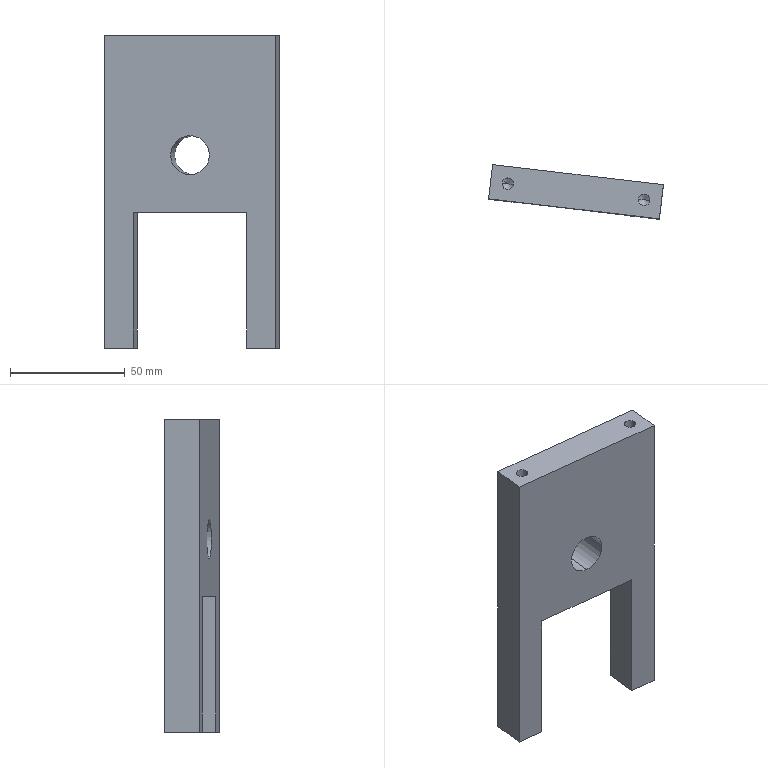Component | SolidWorks | 8TC-A17001-90-01PressureRollerSidePlate1-1 | 1 solid | 28 faces | box 76.24 x 23.65 x 136.2 mm | volume 103614 mm3 | cylinder 10 | plane 10 | cone 8 | commonest cylinder face diameters 5 x8 17 x2 | material #45
build123d program:
from build123d import *

# Parameters (mm, degrees)
SKETCH1_W                  = 75
SKETCH1_H                  = 77
BOSS_EXTRUDE1_DEPTH        = 7.5
SKETCH23_W                 = 12.5
SKETCH23_H                 = 15
BOSS_EXTRUDE4_DEPTH        = 59.2
M6_TAPPED_HOLE2_D          = 5
M6_TAPPED_HOLE2_DEPTH      = 25
M6_TAPPED_HOLE2_TIP        = 1.502
M6_TAPPED_HOLE1_D          = 5
M6_TAPPED_HOLE1_DEPTH      = 20
M6_TAPPED_HOLE1_TIP        = 1.502
F_15_0_15_DIAMETER_HOLE1_D = 17


with BuildPart() as part:
    # Sketch1 → Boss-Extrude1 (new, symmetric)
    with BuildSketch(Plane(origin=(0, 0, 0), x_dir=(1, 0, 0), z_dir=(0, 1, 0))):
        Rectangle(SKETCH1_W, SKETCH1_H)
    extrude(amount=BOSS_EXTRUDE1_DEPTH, both=True)

    # Sketch23 → Boss-Extrude4 (add)
    with BuildSketch(Plane.XY.offset(38.5)):
        with Locations((-31.25, 0)):
            Rectangle(SKETCH23_W, SKETCH23_H)
        with Locations((31.25, 0)):
            Rectangle(SKETCH23_W, SKETCH23_H)
    extrude(amount=BOSS_EXTRUDE4_DEPTH)

    # M6 Tapped Hole2
    with Locations(Plane.XY.offset(97.7)):
        with Locations((-30, 0), (30, 0)):
            Hole(M6_TAPPED_HOLE2_D / 2, depth=M6_TAPPED_HOLE2_DEPTH)
            with Locations((0, 0, -(M6_TAPPED_HOLE2_DEPTH + M6_TAPPED_HOLE2_TIP / 2))):  # 118° drill point
                Cone(0, M6_TAPPED_HOLE2_D / 2, M6_TAPPED_HOLE2_TIP, mode=Mode.SUBTRACT)

    # M6 Tapped Hole1
    with Locations(Plane(origin=(0, 0, -38.5), x_dir=(-1, 0, 0), z_dir=(0, 0, -1))):
        with Locations((-30, 0), (30, 0)):
            Hole(M6_TAPPED_HOLE1_D / 2, depth=M6_TAPPED_HOLE1_DEPTH)
            with Locations((0, 0, -(M6_TAPPED_HOLE1_DEPTH + M6_TAPPED_HOLE1_TIP / 2))):  # 118° drill point
                Cone(0, M6_TAPPED_HOLE1_D / 2, M6_TAPPED_HOLE1_TIP, mode=Mode.SUBTRACT)

    # 15.0 _15_ Diameter Hole1 (through all)
    with Locations(Plane(origin=(0, 7.5, 0), x_dir=(1, 0, 0), z_dir=(0, 1, 0))):
        with Locations((0, -13.5)):
            Hole(F_15_0_15_DIAMETER_HOLE1_D / 2)


solid = part.part

# Placed as in the assembly
solid = solid.moved(Location((-0.2049, -94, -38.5), (-180, 0, -173.3)))
STEP:
#1=COLOUR_RGB('',0.7922,0.8196,0.9333);
#2=FILL_AREA_STYLE_COLOUR('',#1);
#3=FILL_AREA_STYLE('',(#2));
#4=SURFACE_STYLE_FILL_AREA(#3);
#5=SURFACE_SIDE_STYLE('',(#4));
#6=SURFACE_STYLE_USAGE(.BOTH.,#5);
#7=PRESENTATION_STYLE_ASSIGNMENT((#6));
#8=CARTESIAN_POINT('',(-0.04251,-3.994,-1.713));
#9=VERTEX_POINT('',#8);
#10=CARTESIAN_POINT('',(-0.04251,-3.994,-2.382));
#11=VERTEX_POINT('',#10);
#12=CARTESIAN_POINT('',(-0.04251,-3.994,-2.047));
#13=DIRECTION('',(0.1167,0.9932,-0.));
#14=DIRECTION('',(0.,0.,-1.));
#15=AXIS2_PLACEMENT_3D('',#12,#13,#14);
#16=CIRCLE('',#15,0.3346);
#17=EDGE_CURVE('',#9,#11,#16,.T.);
#18=ORIENTED_EDGE('',*,*,#17,.F.);
#19=CARTESIAN_POINT('',(0.02638,-3.408,-1.713));
#20=VERTEX_POINT('',#19);
#21=CARTESIAN_POINT('',(0.02638,-3.408,-1.713));
#22=DIRECTION('',(0.1167,0.9932,-0.));
#23=VECTOR('',#22,39.37);
#24=LINE('',#21,#23);
#25=EDGE_CURVE('',#9,#20,#24,.T.);
#26=ORIENTED_EDGE('',*,*,#25,.T.);
#27=CARTESIAN_POINT('',(0.02638,-3.408,-2.382));
#28=VERTEX_POINT('',#27);
#29=CARTESIAN_POINT('',(0.02638,-3.408,-2.047));
#30=DIRECTION('',(0.1167,0.9932,-0.));
#31=DIRECTION('',(0.,0.,-1.));
#32=AXIS2_PLACEMENT_3D('',#29,#30,#31);
#33=CIRCLE('',#32,0.3346);
#34=EDGE_CURVE('',#20,#28,#33,.T.);
#35=ORIENTED_EDGE('',*,*,#34,.T.);
#36=CARTESIAN_POINT('',(0.02638,-3.408,-2.382));
#37=DIRECTION('',(0.1167,0.9932,-0.));
#38=VECTOR('',#37,39.37);
#39=LINE('',#36,#38);
#40=EDGE_CURVE('',#11,#28,#39,.T.);
#41=ORIENTED_EDGE('',*,*,#40,.F.);
#42=EDGE_LOOP('',(#18,#26,#35,#41));
#43=FACE_OUTER_BOUND('',#42,.T.);
#44=CARTESIAN_POINT('',(0.02638,-3.408,-2.047));
#45=DIRECTION('',(0.1167,0.9932,-0.));
#46=DIRECTION('',(0.,0.,-1.));
#47=AXIS2_PLACEMENT_3D('',#44,#45,#46);
#48=CYLINDRICAL_SURFACE('',#47,0.3346);
#49=ADVANCED_FACE('',(#43),#48,.F.);
#50=CARTESIAN_POINT('',(-1.279,-3.552,-0.7874));
#51=VERTEX_POINT('',#50);
#52=CARTESIAN_POINT('',(-1.083,-3.574,-0.7874));
#53=VERTEX_POINT('',#52);
#54=CARTESIAN_POINT('',(-1.181,-3.563,-0.7874));
#55=DIRECTION('',(-0.,0.,1.));
#56=DIRECTION('',(0.9932,-0.1167,0.));
#57=AXIS2_PLACEMENT_3D('',#54,#55,#56);
#58=CIRCLE('',#57,0.09843);
#59=EDGE_CURVE('',#51,#53,#58,.T.);
#60=ORIENTED_EDGE('',*,*,#59,.F.);
#61=CARTESIAN_POINT('',(-1.279,-3.552,-0.));
#62=VERTEX_POINT('',#61);
#63=CARTESIAN_POINT('',(-1.279,-3.552,-0.));
#64=DIRECTION('',(-0.,0.,1.));
#65=VECTOR('',#64,39.37);
#66=LINE('',#63,#65);
#67=EDGE_CURVE('',#51,#62,#66,.T.);
#68=ORIENTED_EDGE('',*,*,#67,.T.);
#69=CARTESIAN_POINT('',(-1.083,-3.574,0.));
#70=VERTEX_POINT('',#69);
#71=CARTESIAN_POINT('',(-1.181,-3.563,0.));
#72=DIRECTION('',(-0.,0.,1.));
#73=DIRECTION('',(0.9932,-0.1167,0.));
#74=AXIS2_PLACEMENT_3D('',#71,#72,#73);
#75=CIRCLE('',#74,0.09843);
#76=EDGE_CURVE('',#62,#70,#75,.T.);
#77=ORIENTED_EDGE('',*,*,#76,.T.);
#78=CARTESIAN_POINT('',(-1.083,-3.574,0.));
#79=DIRECTION('',(-0.,0.,1.));
#80=VECTOR('',#79,39.37);
#81=LINE('',#78,#80);
#82=EDGE_CURVE('',#53,#70,#81,.T.);
#83=ORIENTED_EDGE('',*,*,#82,.F.);
#84=EDGE_LOOP('',(#60,#68,#77,#83));
#85=FACE_OUTER_BOUND('',#84,.T.);
#86=CARTESIAN_POINT('',(-1.181,-3.563,0.));
#87=DIRECTION('',(-0.,0.,1.));
#88=DIRECTION('',(0.9932,-0.1167,0.));
#89=AXIS2_PLACEMENT_3D('',#86,#87,#88);
#90=CYLINDRICAL_SURFACE('',#89,0.09843);
#91=ADVANCED_FACE('',(#85),#90,.F.);
#92=CARTESIAN_POINT('',(-1.181,-3.563,-0.8465));
#93=VERTEX_POINT('',#92);
#94=CARTESIAN_POINT('',(-1.083,-3.574,-0.7874));
#95=DIRECTION('',(0.8513,-0.1,0.515));
#96=VECTOR('',#95,39.37);
#97=LINE('',#94,#96);
#98=EDGE_CURVE('',#93,#53,#97,.T.);
#99=ORIENTED_EDGE('',*,*,#98,.F.);
#100=CARTESIAN_POINT('',(-1.279,-3.552,-0.7874));
#101=DIRECTION('',(-0.8513,0.1,0.515));
#102=VECTOR('',#101,39.37);
#103=LINE('',#100,#102);
#104=EDGE_CURVE('',#93,#51,#103,.T.);
#105=ORIENTED_EDGE('',*,*,#104,.T.);
#106=ORIENTED_EDGE('',*,*,#59,.T.);
#107=EDGE_LOOP('',(#99,#105,#106));
#108=FACE_OUTER_BOUND('',#107,.T.);
#109=CARTESIAN_POINT('',(-1.181,-3.563,-0.7874));
#110=DIRECTION('',(-0.,0.,1.));
#111=DIRECTION('',(0.9932,-0.1167,0.));
#112=AXIS2_PLACEMENT_3D('',#109,#110,#111);
#113=CONICAL_SURFACE('',#112,0.09843,1.03);
#114=ADVANCED_FACE('',(#108),#113,.F.);
#115=CARTESIAN_POINT('',(1.067,-3.827,-0.7874));
#116=VERTEX_POINT('',#115);
#117=CARTESIAN_POINT('',(1.263,-3.85,-0.7874));
#118=VERTEX_POINT('',#117);
#119=CARTESIAN_POINT('',(1.165,-3.839,-0.7874));
#120=DIRECTION('',(-0.,0.,1.));
#121=DIRECTION('',(0.9932,-0.1167,0.));
#122=AXIS2_PLACEMENT_3D('',#119,#120,#121);
#123=CIRCLE('',#122,0.09843);
#124=EDGE_CURVE('',#116,#118,#123,.T.);
#125=ORIENTED_EDGE('',*,*,#124,.F.);
#126=CARTESIAN_POINT('',(1.067,-3.827,-0.));
#127=VERTEX_POINT('',#126);
#128=CARTESIAN_POINT('',(1.067,-3.827,-0.));
#129=DIRECTION('',(-0.,0.,1.));
#130=VECTOR('',#129,39.37);
#131=LINE('',#128,#130);
#132=EDGE_CURVE('',#116,#127,#131,.T.);
#133=ORIENTED_EDGE('',*,*,#132,.T.);
#134=CARTESIAN_POINT('',(1.263,-3.85,0.));
#135=VERTEX_POINT('',#134);
#136=CARTESIAN_POINT('',(1.165,-3.839,0.));
#137=DIRECTION('',(-0.,0.,1.));
#138=DIRECTION('',(0.9932,-0.1167,0.));
#139=AXIS2_PLACEMENT_3D('',#136,#137,#138);
#140=CIRCLE('',#139,0.09843);
#141=EDGE_CURVE('',#127,#135,#140,.T.);
#142=ORIENTED_EDGE('',*,*,#141,.T.);
#143=CARTESIAN_POINT('',(1.263,-3.85,0.));
#144=DIRECTION('',(-0.,0.,1.));
#145=VECTOR('',#144,39.37);
#146=LINE('',#143,#145);
#147=EDGE_CURVE('',#118,#135,#146,.T.);
#148=ORIENTED_EDGE('',*,*,#147,.F.);
#149=EDGE_LOOP('',(#125,#133,#142,#148));
#150=FACE_OUTER_BOUND('',#149,.T.);
#151=CARTESIAN_POINT('',(1.165,-3.839,0.));
#152=DIRECTION('',(-0.,0.,1.));
#153=DIRECTION('',(0.9932,-0.1167,0.));
#154=AXIS2_PLACEMENT_3D('',#151,#152,#153);
#155=CYLINDRICAL_SURFACE('',#154,0.09843);
#156=ADVANCED_FACE('',(#150),#155,.F.);
#157=CARTESIAN_POINT('',(1.165,-3.839,-0.8465));
#158=VERTEX_POINT('',#157);
#159=CARTESIAN_POINT('',(1.263,-3.85,-0.7874));
#160=DIRECTION('',(0.8513,-0.1,0.515));
#161=VECTOR('',#160,39.37);
#162=LINE('',#159,#161);
#163=EDGE_CURVE('',#158,#118,#162,.T.);
#164=ORIENTED_EDGE('',*,*,#163,.F.);
#165=CARTESIAN_POINT('',(1.067,-3.827,-0.7874));
#166=DIRECTION('',(-0.8513,0.1,0.515));
#167=VECTOR('',#166,39.37);
#168=LINE('',#165,#167);
#169=EDGE_CURVE('',#158,#116,#168,.T.);
#170=ORIENTED_EDGE('',*,*,#169,.T.);
#171=ORIENTED_EDGE('',*,*,#124,.T.);
#172=EDGE_LOOP('',(#164,#170,#171));
#173=FACE_OUTER_BOUND('',#172,.T.);
#174=CARTESIAN_POINT('',(1.165,-3.839,-0.7874));
#175=DIRECTION('',(-0.,0.,1.));
#176=DIRECTION('',(0.9932,-0.1167,0.));
#177=AXIS2_PLACEMENT_3D('',#174,#175,#176);
#178=CONICAL_SURFACE('',#177,0.09843,1.03);
#179=ADVANCED_FACE('',(#173),#178,.F.);
#180=CARTESIAN_POINT('',(1.263,-3.85,-4.378));
#181=VERTEX_POINT('',#180);
#182=CARTESIAN_POINT('',(1.067,-3.827,-4.378));
#183=VERTEX_POINT('',#182);
#184=CARTESIAN_POINT('',(1.165,-3.839,-4.378));
#185=DIRECTION('',(0.,-0.,-1.));
#186=DIRECTION('',(-0.9932,0.1167,0.));
#187=AXIS2_PLACEMENT_3D('',#184,#185,#186);
#188=CIRCLE('',#187,0.09843);
#189=EDGE_CURVE('',#181,#183,#188,.T.);
#190=ORIENTED_EDGE('',*,*,#189,.F.);
#191=CARTESIAN_POINT('',(1.263,-3.85,-5.362));
#192=VERTEX_POINT('',#191);
#193=CARTESIAN_POINT('',(1.263,-3.85,-5.362));
#194=DIRECTION('',(0.,-0.,-1.));
#195=VECTOR('',#194,39.37);
#196=LINE('',#193,#195);
#197=EDGE_CURVE('',#181,#192,#196,.T.);
#198=ORIENTED_EDGE('',*,*,#197,.T.);
#199=CARTESIAN_POINT('',(1.067,-3.827,-5.362));
#200=VERTEX_POINT('',#199);
#201=CARTESIAN_POINT('',(1.165,-3.839,-5.362));
#202=DIRECTION('',(0.,-0.,-1.));
#203=DIRECTION('',(-0.9932,0.1167,0.));
#204=AXIS2_PLACEMENT_3D('',#201,#202,#203);
#205=CIRCLE('',#204,0.09843);
#206=EDGE_CURVE('',#192,#200,#205,.T.);
#207=ORIENTED_EDGE('',*,*,#206,.T.);
#208=CARTESIAN_POINT('',(1.067,-3.827,-5.362));
#209=DIRECTION('',(0.,-0.,-1.));
#210=VECTOR('',#209,39.37);
#211=LINE('',#208,#210);
#212=EDGE_CURVE('',#183,#200,#211,.T.);
#213=ORIENTED_EDGE('',*,*,#212,.F.);
#214=EDGE_LOOP('',(#190,#198,#207,#213));
#215=FACE_OUTER_BOUND('',#214,.T.);
#216=CARTESIAN_POINT('',(1.165,-3.839,-5.362));
#217=DIRECTION('',(0.,-0.,-1.));
#218=DIRECTION('',(-0.9932,0.1167,0.));
#219=AXIS2_PLACEMENT_3D('',#216,#217,#218);
#220=CYLINDRICAL_SURFACE('',#219,0.09843);
#221=ADVANCED_FACE('',(#215),#220,.F.);
#222=CARTESIAN_POINT('',(1.165,-3.839,-4.319));
#223=VERTEX_POINT('',#222);
#224=CARTESIAN_POINT('',(1.067,-3.827,-4.378));
#225=DIRECTION('',(-0.8513,0.1,-0.515));
#226=VECTOR('',#225,39.37);
#227=LINE('',#224,#226);
#228=EDGE_CURVE('',#223,#183,#227,.T.);
#229=ORIENTED_EDGE('',*,*,#228,.F.);
#230=CARTESIAN_POINT('',(1.263,-3.85,-4.378));
#231=DIRECTION('',(0.8513,-0.1,-0.515));
#232=VECTOR('',#231,39.37);
#233=LINE('',#230,#232);
#234=EDGE_CURVE('',#223,#181,#233,.T.);
#235=ORIENTED_EDGE('',*,*,#234,.T.);
#236=ORIENTED_EDGE('',*,*,#189,.T.);
#237=EDGE_LOOP('',(#229,#235,#236));
#238=FACE_OUTER_BOUND('',#237,.T.);
#239=CARTESIAN_POINT('',(1.165,-3.839,-4.378));
#240=DIRECTION('',(0.,-0.,-1.));
#241=DIRECTION('',(-0.9932,0.1167,0.));
#242=AXIS2_PLACEMENT_3D('',#239,#240,#241);
#243=CONICAL_SURFACE('',#242,0.09843,1.03);
#244=ADVANCED_FACE('',(#238),#243,.F.);
#245=CARTESIAN_POINT('',(-1.083,-3.574,-4.378));
#246=VERTEX_POINT('',#245);
#247=CARTESIAN_POINT('',(-1.279,-3.552,-4.378));
#248=VERTEX_POINT('',#247);
#249=CARTESIAN_POINT('',(-1.181,-3.563,-4.378));
#250=DIRECTION('',(0.,-0.,-1.));
#251=DIRECTION('',(-0.9932,0.1167,0.));
#252=AXIS2_PLACEMENT_3D('',#249,#250,#251);
#253=CIRCLE('',#252,0.09843);
#254=EDGE_CURVE('',#246,#248,#253,.T.);
#255=ORIENTED_EDGE('',*,*,#254,.F.);
#256=CARTESIAN_POINT('',(-1.083,-3.574,-5.362));
#257=VERTEX_POINT('',#256);
#258=CARTESIAN_POINT('',(-1.083,-3.574,-5.362));
#259=DIRECTION('',(0.,-0.,-1.));
#260=VECTOR('',#259,39.37);
#261=LINE('',#258,#260);
#262=EDGE_CURVE('',#246,#257,#261,.T.);
#263=ORIENTED_EDGE('',*,*,#262,.T.);
#264=CARTESIAN_POINT('',(-1.279,-3.552,-5.362));
#265=VERTEX_POINT('',#264);
#266=CARTESIAN_POINT('',(-1.181,-3.563,-5.362));
#267=DIRECTION('',(0.,-0.,-1.));
#268=DIRECTION('',(-0.9932,0.1167,0.));
#269=AXIS2_PLACEMENT_3D('',#266,#267,#268);
#270=CIRCLE('',#269,0.09843);
#271=EDGE_CURVE('',#257,#265,#270,.T.);
#272=ORIENTED_EDGE('',*,*,#271,.T.);
#273=CARTESIAN_POINT('',(-1.279,-3.552,-5.362));
#274=DIRECTION('',(0.,-0.,-1.));
#275=VECTOR('',#274,39.37);
#276=LINE('',#273,#275);
#277=EDGE_CURVE('',#248,#265,#276,.T.);
#278=ORIENTED_EDGE('',*,*,#277,.F.);
#279=EDGE_LOOP('',(#255,#263,#272,#278));
#280=FACE_OUTER_BOUND('',#279,.T.);
#281=CARTESIAN_POINT('',(-1.181,-3.563,-5.362));
#282=DIRECTION('',(0.,-0.,-1.));
#283=DIRECTION('',(-0.9932,0.1167,0.));
#284=AXIS2_PLACEMENT_3D('',#281,#282,#283);
#285=CYLINDRICAL_SURFACE('',#284,0.09843);
#286=ADVANCED_FACE('',(#280),#285,.F.);
#287=CARTESIAN_POINT('',(-1.181,-3.563,-4.319));
#288=VERTEX_POINT('',#287);
#289=CARTESIAN_POINT('',(-1.279,-3.552,-4.378));
#290=DIRECTION('',(-0.8513,0.1,-0.515));
#291=VECTOR('',#290,39.37);
#292=LINE('',#289,#291);
#293=EDGE_CURVE('',#288,#248,#292,.T.);
#294=ORIENTED_EDGE('',*,*,#293,.F.);
#295=CARTESIAN_POINT('',(-1.083,-3.574,-4.378));
#296=DIRECTION('',(0.8513,-0.1,-0.515));
#297=VECTOR('',#296,39.37);
#298=LINE('',#295,#297);
#299=EDGE_CURVE('',#288,#246,#298,.T.);
#300=ORIENTED_EDGE('',*,*,#299,.T.);
#301=ORIENTED_EDGE('',*,*,#254,.T.);
#302=EDGE_LOOP('',(#294,#300,#301));
#303=FACE_OUTER_BOUND('',#302,.T.);
#304=CARTESIAN_POINT('',(-1.181,-3.563,-4.378));
#305=DIRECTION('',(0.,-0.,-1.));
#306=DIRECTION('',(-0.9932,0.1167,0.));
#307=AXIS2_PLACEMENT_3D('',#304,#305,#306);
#308=CONICAL_SURFACE('',#307,0.09843,1.03);
#309=ADVANCED_FACE('',(#303),#308,.F.);
#310=CARTESIAN_POINT('',(-0.9511,-3.293,-3.031));
#311=VERTEX_POINT('',#310);
#312=CARTESIAN_POINT('',(-1.02,-3.879,-3.031));
#313=VERTEX_POINT('',#312);
#314=CARTESIAN_POINT('',(-0.9511,-3.293,-3.031));
#315=DIRECTION('',(-0.1167,-0.9932,0.));
#316=VECTOR('',#315,39.37);
#317=LINE('',#314,#316);
#318=EDGE_CURVE('',#311,#313,#317,.T.);
#319=ORIENTED_EDGE('',*,*,#318,.F.);
#320=CARTESIAN_POINT('',(1.004,-3.522,-3.031));
#321=VERTEX_POINT('',#320);
#322=CARTESIAN_POINT('',(1.493,-3.58,-3.031));
#323=DIRECTION('',(-0.9932,0.1167,-0.));
#324=VECTOR('',#323,39.37);
#325=LINE('',#322,#324);
#326=EDGE_CURVE('',#321,#311,#325,.T.);
#327=ORIENTED_EDGE('',*,*,#326,.F.);
#328=CARTESIAN_POINT('',(0.935,-4.109,-3.031));
#329=VERTEX_POINT('',#328);
#330=CARTESIAN_POINT('',(1.004,-3.522,-3.031));
#331=DIRECTION('',(0.1167,0.9932,-0.));
#332=VECTOR('',#331,39.37);
#333=LINE('',#330,#332);
#334=EDGE_CURVE('',#329,#321,#333,.T.);
#335=ORIENTED_EDGE('',*,*,#334,.F.);
#336=CARTESIAN_POINT('',(1.424,-4.166,-3.031));
#337=DIRECTION('',(-0.9932,0.1167,-0.));
#338=VECTOR('',#337,39.37);
#339=LINE('',#336,#338);
#340=EDGE_CURVE('',#329,#313,#339,.T.);
#341=ORIENTED_EDGE('',*,*,#340,.T.);
#342=EDGE_LOOP('',(#319,#327,#335,#341));
#343=FACE_OUTER_BOUND('',#342,.T.);
#344=CARTESIAN_POINT('',(1.493,-3.58,-3.031));
#345=DIRECTION('',(-0.,0.,1.));
#346=DIRECTION('',(0.9932,-0.1167,0.));
#347=AXIS2_PLACEMENT_3D('',#344,#345,#346);
#348=PLANE('',#347);
#349=ADVANCED_FACE('',(#343),#348,.F.);
#350=CARTESIAN_POINT('',(-1.509,-3.822,-5.362));
#351=VERTEX_POINT('',#350);
#352=CARTESIAN_POINT('',(-1.509,-3.822,0.));
#353=VERTEX_POINT('',#352);
#354=CARTESIAN_POINT('',(-1.509,-3.822,0.));
#355=DIRECTION('',(0.,-0.,1.));
#356=VECTOR('',#355,39.37);
#357=LINE('',#354,#356);
#358=EDGE_CURVE('',#351,#353,#357,.T.);
#359=ORIENTED_EDGE('',*,*,#358,.T.);
#360=CARTESIAN_POINT('',(-1.44,-3.235,0.));
#361=VERTEX_POINT('',#360);
#362=CARTESIAN_POINT('',(-1.44,-3.235,0.));
#363=DIRECTION('',(-0.1167,-0.9932,0.));
#364=VECTOR('',#363,39.37);
#365=LINE('',#362,#364);
#366=EDGE_CURVE('',#361,#353,#365,.T.);
#367=ORIENTED_EDGE('',*,*,#366,.F.);
#368=CARTESIAN_POINT('',(-1.44,-3.235,-5.362));
#369=VERTEX_POINT('',#368);
#370=CARTESIAN_POINT('',(-1.44,-3.235,0.));
#371=DIRECTION('',(0.,-0.,1.));
#372=VECTOR('',#371,39.37);
#373=LINE('',#370,#372);
#374=EDGE_CURVE('',#369,#361,#373,.T.);
#375=ORIENTED_EDGE('',*,*,#374,.F.);
#376=CARTESIAN_POINT('',(-1.44,-3.235,-5.362));
#377=DIRECTION('',(0.1167,0.9932,-0.));
#378=VECTOR('',#377,39.37);
#379=LINE('',#376,#378);
#380=EDGE_CURVE('',#351,#369,#379,.T.);
#381=ORIENTED_EDGE('',*,*,#380,.F.);
#382=EDGE_LOOP('',(#359,#367,#375,#381));
#383=FACE_OUTER_BOUND('',#382,.T.);
#384=CARTESIAN_POINT('',(-1.44,-3.235,0.));
#385=DIRECTION('',(0.9932,-0.1167,-0.));
#386=DIRECTION('',(-0.,0.,-1.));
#387=AXIS2_PLACEMENT_3D('',#384,#385,#386);
#388=PLANE('',#387);
#389=ADVANCED_FACE('',(#383),#388,.F.);
#390=CARTESIAN_POINT('',(-1.181,-3.563,0.));
#391=DIRECTION('',(-0.,0.,1.));
#392=DIRECTION('',(0.9932,-0.1167,0.));
#393=AXIS2_PLACEMENT_3D('',#390,#391,#392);
#394=CIRCLE('',#393,0.09843);
#395=EDGE_CURVE('',#70,#62,#394,.T.);
#396=ORIENTED_EDGE('',*,*,#395,.F.);
#397=ORIENTED_EDGE('',*,*,#76,.F.);
#398=EDGE_LOOP('',(#396,#397));
#399=FACE_BOUND('',#398,.T.);
#400=CARTESIAN_POINT('',(1.165,-3.839,0.));
#401=DIRECTION('',(-0.,0.,1.));
#402=DIRECTION('',(0.9932,-0.1167,0.));
#403=AXIS2_PLACEMENT_3D('',#400,#401,#402);
#404=CIRCLE('',#403,0.09843);
#405=EDGE_CURVE('',#135,#127,#404,.T.);
#406=ORIENTED_EDGE('',*,*,#405,.F.);
#407=ORIENTED_EDGE('',*,*,#141,.F.);
#408=EDGE_LOOP('',(#406,#407));
#409=FACE_BOUND('',#408,.T.);
#410=CARTESIAN_POINT('',(1.424,-4.166,0.));
#411=VERTEX_POINT('',#410);
#412=CARTESIAN_POINT('',(1.424,-4.166,0.));
#413=DIRECTION('',(0.9932,-0.1167,0.));
#414=VECTOR('',#413,39.37);
#415=LINE('',#412,#414);
#416=EDGE_CURVE('',#353,#411,#415,.T.);
#417=ORIENTED_EDGE('',*,*,#416,.T.);
#418=CARTESIAN_POINT('',(1.493,-3.58,0.));
#419=VERTEX_POINT('',#418);
#420=CARTESIAN_POINT('',(1.493,-3.58,0.));
#421=DIRECTION('',(-0.1167,-0.9932,0.));
#422=VECTOR('',#421,39.37);
#423=LINE('',#420,#422);
#424=EDGE_CURVE('',#419,#411,#423,.T.);
#425=ORIENTED_EDGE('',*,*,#424,.F.);
#426=CARTESIAN_POINT('',(1.493,-3.58,0.));
#427=DIRECTION('',(0.9932,-0.1167,0.));
#428=VECTOR('',#427,39.37);
#429=LINE('',#426,#428);
#430=EDGE_CURVE('',#361,#419,#429,.T.);
#431=ORIENTED_EDGE('',*,*,#430,.F.);
#432=ORIENTED_EDGE('',*,*,#366,.T.);
#433=EDGE_LOOP('',(#417,#425,#431,#432));
#434=FACE_OUTER_BOUND('',#433,.T.);
#435=CARTESIAN_POINT('',(1.493,-3.58,0.));
#436=DIRECTION('',(0.,-0.,-1.));
#437=DIRECTION('',(-0.9932,0.1167,-0.));
#438=AXIS2_PLACEMENT_3D('',#435,#436,#437);
#439=PLANE('',#438);
#440=ADVANCED_FACE('',(#399,#409,#434),#439,.F.);
#441=CARTESIAN_POINT('',(1.424,-4.166,-5.362));
#442=VERTEX_POINT('',#441);
#443=CARTESIAN_POINT('',(1.424,-4.166,0.));
#444=DIRECTION('',(-0.,0.,-1.));
#445=VECTOR('',#444,39.37);
#446=LINE('',#443,#445);
#447=EDGE_CURVE('',#411,#442,#446,.T.);
#448=ORIENTED_EDGE('',*,*,#447,.T.);
#449=CARTESIAN_POINT('',(1.493,-3.58,-5.362));
#450=VERTEX_POINT('',#449);
#451=CARTESIAN_POINT('',(1.493,-3.58,-5.362));
#452=DIRECTION('',(-0.1167,-0.9932,0.));
#453=VECTOR('',#452,39.37);
#454=LINE('',#451,#453);
#455=EDGE_CURVE('',#450,#442,#454,.T.);
#456=ORIENTED_EDGE('',*,*,#455,.F.);
#457=CARTESIAN_POINT('',(1.493,-3.58,0.));
#458=DIRECTION('',(-0.,0.,-1.));
#459=VECTOR('',#458,39.37);
#460=LINE('',#457,#459);
#461=EDGE_CURVE('',#419,#450,#460,.T.);
#462=ORIENTED_EDGE('',*,*,#461,.F.);
#463=ORIENTED_EDGE('',*,*,#424,.T.);
#464=EDGE_LOOP('',(#448,#456,#462,#463));
#465=FACE_OUTER_BOUND('',#464,.T.);
#466=CARTESIAN_POINT('',(1.493,-3.58,0.));
#467=DIRECTION('',(-0.9932,0.1167,0.));
#468=DIRECTION('',(0.,-0.,1.));
#469=AXIS2_PLACEMENT_3D('',#466,#467,#468);
#470=PLANE('',#469);
#471=ADVANCED_FACE('',(#465),#470,.F.);
#472=CARTESIAN_POINT('',(0.02638,-3.408,-2.047));
#473=DIRECTION('',(0.1167,0.9932,-0.));
#474=DIRECTION('',(0.,0.,-1.));
#475=AXIS2_PLACEMENT_3D('',#472,#473,#474);
#476=CIRCLE('',#475,0.3346);
#477=EDGE_CURVE('',#28,#20,#476,.T.);
#478=ORIENTED_EDGE('',*,*,#477,.F.);
#479=ORIENTED_EDGE('',*,*,#34,.F.);
#480=EDGE_LOOP('',(#478,#479));
#481=FACE_BOUND('',#480,.T.);
#482=ORIENTED_EDGE('',*,*,#374,.T.);
#483=ORIENTED_EDGE('',*,*,#430,.T.);
#484=ORIENTED_EDGE('',*,*,#461,.T.);
#485=CARTESIAN_POINT('',(1.004,-3.522,-5.362));
#486=VERTEX_POINT('',#485);
#487=CARTESIAN_POINT('',(1.493,-3.58,-5.362));
#488=DIRECTION('',(0.9932,-0.1167,0.));
#489=VECTOR('',#488,39.37);
#490=LINE('',#487,#489);
#491=EDGE_CURVE('',#486,#450,#490,.T.);
#492=ORIENTED_EDGE('',*,*,#491,.F.);
#493=CARTESIAN_POINT('',(1.004,-3.522,-5.362));
#494=DIRECTION('',(-0.,0.,1.));
#495=VECTOR('',#494,39.37);
#496=LINE('',#493,#495);
#497=EDGE_CURVE('',#486,#321,#496,.T.);
#498=ORIENTED_EDGE('',*,*,#497,.T.);
#499=ORIENTED_EDGE('',*,*,#326,.T.);
#500=CARTESIAN_POINT('',(-0.9511,-3.293,-5.362));
#501=VERTEX_POINT('',#500);
#502=CARTESIAN_POINT('',(-0.9511,-3.293,-5.362));
#503=DIRECTION('',(-0.,0.,1.));
#504=VECTOR('',#503,39.37);
#505=LINE('',#502,#504);
#506=EDGE_CURVE('',#501,#311,#505,.T.);
#507=ORIENTED_EDGE('',*,*,#506,.F.);
#508=CARTESIAN_POINT('',(-1.44,-3.235,-5.362));
#509=DIRECTION('',(0.9932,-0.1167,0.));
#510=VECTOR('',#509,39.37);
#511=LINE('',#508,#510);
#512=EDGE_CURVE('',#369,#501,#511,.T.);
#513=ORIENTED_EDGE('',*,*,#512,.F.);
#514=EDGE_LOOP('',(#482,#483,#484,#492,#498,#499,#507,#513));
#515=FACE_OUTER_BOUND('',#514,.T.);
#516=CARTESIAN_POINT('',(0.02638,-3.408,-1.516));
#517=DIRECTION('',(0.1167,0.9932,-0.));
#518=DIRECTION('',(0.,-0.,-1.));
#519=AXIS2_PLACEMENT_3D('',#516,#517,#518);
#520=PLANE('',#519);
#521=ADVANCED_FACE('',(#481,#515),#520,.T.);
#522=CARTESIAN_POINT('',(-0.04251,-3.994,-2.047));
#523=DIRECTION('',(0.1167,0.9932,-0.));
#524=DIRECTION('',(0.,0.,-1.));
#525=AXIS2_PLACEMENT_3D('',#522,#523,#524);
#526=CIRCLE('',#525,0.3346);
#527=EDGE_CURVE('',#11,#9,#526,.T.);
#528=ORIENTED_EDGE('',*,*,#527,.T.);
#529=ORIENTED_EDGE('',*,*,#17,.T.);
#530=EDGE_LOOP('',(#528,#529));
#531=FACE_BOUND('',#530,.T.);
#532=ORIENTED_EDGE('',*,*,#358,.F.);
#533=CARTESIAN_POINT('',(-1.02,-3.879,-5.362));
#534=VERTEX_POINT('',#533);
#535=CARTESIAN_POINT('',(-1.509,-3.822,-5.362));
#536=DIRECTION('',(-0.9932,0.1167,-0.));
#537=VECTOR('',#536,39.37);
#538=LINE('',#535,#537);
#539=EDGE_CURVE('',#534,#351,#538,.T.);
#540=ORIENTED_EDGE('',*,*,#539,.F.);
#541=CARTESIAN_POINT('',(-1.02,-3.879,-5.362));
#542=DIRECTION('',(-0.,0.,1.));
#543=VECTOR('',#542,39.37);
#544=LINE('',#541,#543);
#545=EDGE_CURVE('',#534,#313,#544,.T.);
#546=ORIENTED_EDGE('',*,*,#545,.T.);
#547=ORIENTED_EDGE('',*,*,#340,.F.);
#548=CARTESIAN_POINT('',(0.935,-4.109,-5.362));
#549=VERTEX_POINT('',#548);
#550=CARTESIAN_POINT('',(0.935,-4.109,-5.362));
#551=DIRECTION('',(-0.,0.,1.));
#552=VECTOR('',#551,39.37);
#553=LINE('',#550,#552);
#554=EDGE_CURVE('',#549,#329,#553,.T.);
#555=ORIENTED_EDGE('',*,*,#554,.F.);
#556=CARTESIAN_POINT('',(1.424,-4.166,-5.362));
#557=DIRECTION('',(-0.9932,0.1167,-0.));
#558=VECTOR('',#557,39.37);
#559=LINE('',#556,#558);
#560=EDGE_CURVE('',#442,#549,#559,.T.);
#561=ORIENTED_EDGE('',*,*,#560,.F.);
#562=ORIENTED_EDGE('',*,*,#447,.F.);
#563=ORIENTED_EDGE('',*,*,#416,.F.);
#564=EDGE_LOOP('',(#532,#540,#546,#547,#555,#561,#562,#563));
#565=FACE_OUTER_BOUND('',#564,.T.);
#566=CARTESIAN_POINT('',(-0.04251,-3.994,-1.516));
#567=DIRECTION('',(0.1167,0.9932,-0.));
#568=DIRECTION('',(0.,-0.,-1.));
#569=AXIS2_PLACEMENT_3D('',#566,#567,#568);
#570=PLANE('',#569);
#571=ADVANCED_FACE('',(#531,#565),#570,.F.);
#572=ORIENTED_EDGE('',*,*,#334,.T.);
#573=ORIENTED_EDGE('',*,*,#497,.F.);
#574=CARTESIAN_POINT('',(1.004,-3.522,-5.362));
#575=DIRECTION('',(0.1167,0.9932,-0.));
#576=VECTOR('',#575,39.37);
#577=LINE('',#574,#576);
#578=EDGE_CURVE('',#549,#486,#577,.T.);
#579=ORIENTED_EDGE('',*,*,#578,.F.);
#580=ORIENTED_EDGE('',*,*,#554,.T.);
#581=EDGE_LOOP('',(#572,#573,#579,#580));
#582=FACE_OUTER_BOUND('',#581,.T.);
#583=CARTESIAN_POINT('',(1.004,-3.522,-5.362));
#584=DIRECTION('',(0.9932,-0.1167,0.));
#585=DIRECTION('',(0.,-0.,-1.));
#586=AXIS2_PLACEMENT_3D('',#583,#584,#585);
#587=PLANE('',#586);
#588=ADVANCED_FACE('',(#582),#587,.F.);
#589=CARTESIAN_POINT('',(1.165,-3.839,-5.362));
#590=DIRECTION('',(0.,-0.,-1.));
#591=DIRECTION('',(-0.9932,0.1167,0.));
#592=AXIS2_PLACEMENT_3D('',#589,#590,#591);
#593=CIRCLE('',#592,0.09843);
#594=EDGE_CURVE('',#200,#192,#593,.T.);
#595=ORIENTED_EDGE('',*,*,#594,.F.);
#596=ORIENTED_EDGE('',*,*,#206,.F.);
#597=EDGE_LOOP('',(#595,#596));
#598=FACE_BOUND('',#597,.T.);
#599=ORIENTED_EDGE('',*,*,#455,.T.);
#600=ORIENTED_EDGE('',*,*,#560,.T.);
#601=ORIENTED_EDGE('',*,*,#578,.T.);
#602=ORIENTED_EDGE('',*,*,#491,.T.);
#603=EDGE_LOOP('',(#599,#600,#601,#602));
#604=FACE_OUTER_BOUND('',#603,.T.);
#605=CARTESIAN_POINT('',(-0.008066,-3.701,-5.362));
#606=DIRECTION('',(0.,-0.,-1.));
#607=DIRECTION('',(-0.9932,0.1167,-0.));
#608=AXIS2_PLACEMENT_3D('',#605,#606,#607);
#609=PLANE('',#608);
#610=ADVANCED_FACE('',(#598,#604),#609,.T.);
#611=ORIENTED_EDGE('',*,*,#318,.T.);
#612=ORIENTED_EDGE('',*,*,#545,.F.);
#613=CARTESIAN_POINT('',(-0.9511,-3.293,-5.362));
#614=DIRECTION('',(-0.1167,-0.9932,0.));
#615=VECTOR('',#614,39.37);
#616=LINE('',#613,#615);
#617=EDGE_CURVE('',#501,#534,#616,.T.);
#618=ORIENTED_EDGE('',*,*,#617,.F.);
#619=ORIENTED_EDGE('',*,*,#506,.T.);
#620=EDGE_LOOP('',(#611,#612,#618,#619));
#621=FACE_OUTER_BOUND('',#620,.T.);
#622=CARTESIAN_POINT('',(-0.9511,-3.293,-5.362));
#623=DIRECTION('',(-0.9932,0.1167,-0.));
#624=DIRECTION('',(-0.,0.,1.));
#625=AXIS2_PLACEMENT_3D('',#622,#623,#624);
#626=PLANE('',#625);
#627=ADVANCED_FACE('',(#621),#626,.F.);
#628=CARTESIAN_POINT('',(-1.181,-3.563,-5.362));
#629=DIRECTION('',(0.,-0.,-1.));
#630=DIRECTION('',(-0.9932,0.1167,0.));
#631=AXIS2_PLACEMENT_3D('',#628,#629,#630);
#632=CIRCLE('',#631,0.09843);
#633=EDGE_CURVE('',#265,#257,#632,.T.);
#634=ORIENTED_EDGE('',*,*,#633,.F.);
#635=ORIENTED_EDGE('',*,*,#271,.F.);
#636=EDGE_LOOP('',(#634,#635));
#637=FACE_BOUND('',#636,.T.);
#638=ORIENTED_EDGE('',*,*,#380,.T.);
#639=ORIENTED_EDGE('',*,*,#512,.T.);
#640=ORIENTED_EDGE('',*,*,#617,.T.);
#641=ORIENTED_EDGE('',*,*,#539,.T.);
#642=EDGE_LOOP('',(#638,#639,#640,#641));
#643=FACE_OUTER_BOUND('',#642,.T.);
#644=CARTESIAN_POINT('',(-0.008066,-3.701,-5.362));
#645=DIRECTION('',(-0.,0.,1.));
#646=DIRECTION('',(0.9932,-0.1167,0.));
#647=AXIS2_PLACEMENT_3D('',#644,#645,#646);
#648=PLANE('',#647);
#649=ADVANCED_FACE('',(#637,#643),#648,.F.);
#650=ORIENTED_EDGE('',*,*,#299,.F.);
#651=ORIENTED_EDGE('',*,*,#293,.T.);
#652=CARTESIAN_POINT('',(-1.181,-3.563,-4.378));
#653=DIRECTION('',(0.,-0.,-1.));
#654=DIRECTION('',(-0.9932,0.1167,0.));
#655=AXIS2_PLACEMENT_3D('',#652,#653,#654);
#656=CIRCLE('',#655,0.09843);
#657=EDGE_CURVE('',#248,#246,#656,.T.);
#658=ORIENTED_EDGE('',*,*,#657,.T.);
#659=EDGE_LOOP('',(#650,#651,#658));
#660=FACE_OUTER_BOUND('',#659,.T.);
#661=CARTESIAN_POINT('',(-1.181,-3.563,-4.378));
#662=DIRECTION('',(0.,-0.,-1.));
#663=DIRECTION('',(-0.9932,0.1167,0.));
#664=AXIS2_PLACEMENT_3D('',#661,#662,#663);
#665=CONICAL_SURFACE('',#664,0.09843,1.03);
#666=ADVANCED_FACE('',(#660),#665,.F.);
#667=ORIENTED_EDGE('',*,*,#262,.F.);
#668=ORIENTED_EDGE('',*,*,#657,.F.);
#669=ORIENTED_EDGE('',*,*,#277,.T.);
#670=ORIENTED_EDGE('',*,*,#633,.T.);
#671=EDGE_LOOP('',(#667,#668,#669,#670));
#672=FACE_OUTER_BOUND('',#671,.T.);
#673=CARTESIAN_POINT('',(-1.181,-3.563,-5.362));
#674=DIRECTION('',(0.,-0.,-1.));
#675=DIRECTION('',(-0.9932,0.1167,0.));
#676=AXIS2_PLACEMENT_3D('',#673,#674,#675);
#677=CYLINDRICAL_SURFACE('',#676,0.09843);
#678=ADVANCED_FACE('',(#672),#677,.F.);
#679=ORIENTED_EDGE('',*,*,#234,.F.);
#680=ORIENTED_EDGE('',*,*,#228,.T.);
#681=CARTESIAN_POINT('',(1.165,-3.839,-4.378));
#682=DIRECTION('',(0.,-0.,-1.));
#683=DIRECTION('',(-0.9932,0.1167,0.));
#684=AXIS2_PLACEMENT_3D('',#681,#682,#683);
#685=CIRCLE('',#684,0.09843);
#686=EDGE_CURVE('',#183,#181,#685,.T.);
#687=ORIENTED_EDGE('',*,*,#686,.T.);
#688=EDGE_LOOP('',(#679,#680,#687));
#689=FACE_OUTER_BOUND('',#688,.T.);
#690=CARTESIAN_POINT('',(1.165,-3.839,-4.378));
#691=DIRECTION('',(0.,-0.,-1.));
#692=DIRECTION('',(-0.9932,0.1167,0.));
#693=AXIS2_PLACEMENT_3D('',#690,#691,#692);
#694=CONICAL_SURFACE('',#693,0.09843,1.03);
#695=ADVANCED_FACE('',(#689),#694,.F.);
#696=ORIENTED_EDGE('',*,*,#197,.F.);
#697=ORIENTED_EDGE('',*,*,#686,.F.);
#698=ORIENTED_EDGE('',*,*,#212,.T.);
#699=ORIENTED_EDGE('',*,*,#594,.T.);
#700=EDGE_LOOP('',(#696,#697,#698,#699));
#701=FACE_OUTER_BOUND('',#700,.T.);
#702=CARTESIAN_POINT('',(1.165,-3.839,-5.362));
#703=DIRECTION('',(0.,-0.,-1.));
#704=DIRECTION('',(-0.9932,0.1167,0.));
#705=AXIS2_PLACEMENT_3D('',#702,#703,#704);
#706=CYLINDRICAL_SURFACE('',#705,0.09843);
#707=ADVANCED_FACE('',(#701),#706,.F.);
#708=ORIENTED_EDGE('',*,*,#169,.F.);
#709=ORIENTED_EDGE('',*,*,#163,.T.);
#710=CARTESIAN_POINT('',(1.165,-3.839,-0.7874));
#711=DIRECTION('',(-0.,0.,1.));
#712=DIRECTION('',(0.9932,-0.1167,0.));
#713=AXIS2_PLACEMENT_3D('',#710,#711,#712);
#714=CIRCLE('',#713,0.09843);
#715=EDGE_CURVE('',#118,#116,#714,.T.);
#716=ORIENTED_EDGE('',*,*,#715,.T.);
#717=EDGE_LOOP('',(#708,#709,#716));
#718=FACE_OUTER_BOUND('',#717,.T.);
#719=CARTESIAN_POINT('',(1.165,-3.839,-0.7874));
#720=DIRECTION('',(-0.,0.,1.));
#721=DIRECTION('',(0.9932,-0.1167,0.));
#722=AXIS2_PLACEMENT_3D('',#719,#720,#721);
#723=CONICAL_SURFACE('',#722,0.09843,1.03);
#724=ADVANCED_FACE('',(#718),#723,.F.);
#725=ORIENTED_EDGE('',*,*,#132,.F.);
#726=ORIENTED_EDGE('',*,*,#715,.F.);
#727=ORIENTED_EDGE('',*,*,#147,.T.);
#728=ORIENTED_EDGE('',*,*,#405,.T.);
#729=EDGE_LOOP('',(#725,#726,#727,#728));
#730=FACE_OUTER_BOUND('',#729,.T.);
#731=CARTESIAN_POINT('',(1.165,-3.839,0.));
#732=DIRECTION('',(-0.,0.,1.));
#733=DIRECTION('',(0.9932,-0.1167,0.));
#734=AXIS2_PLACEMENT_3D('',#731,#732,#733);
#735=CYLINDRICAL_SURFACE('',#734,0.09843);
#736=ADVANCED_FACE('',(#730),#735,.F.);
#737=ORIENTED_EDGE('',*,*,#104,.F.);
#738=ORIENTED_EDGE('',*,*,#98,.T.);
#739=CARTESIAN_POINT('',(-1.181,-3.563,-0.7874));
#740=DIRECTION('',(-0.,0.,1.));
#741=DIRECTION('',(0.9932,-0.1167,0.));
#742=AXIS2_PLACEMENT_3D('',#739,#740,#741);
#743=CIRCLE('',#742,0.09843);
#744=EDGE_CURVE('',#53,#51,#743,.T.);
#745=ORIENTED_EDGE('',*,*,#744,.T.);
#746=EDGE_LOOP('',(#737,#738,#745));
#747=FACE_OUTER_BOUND('',#746,.T.);
#748=CARTESIAN_POINT('',(-1.181,-3.563,-0.7874));
#749=DIRECTION('',(-0.,0.,1.));
#750=DIRECTION('',(0.9932,-0.1167,0.));
#751=AXIS2_PLACEMENT_3D('',#748,#749,#750);
#752=CONICAL_SURFACE('',#751,0.09843,1.03);
#753=ADVANCED_FACE('',(#747),#752,.F.);
#754=ORIENTED_EDGE('',*,*,#67,.F.);
#755=ORIENTED_EDGE('',*,*,#744,.F.);
#756=ORIENTED_EDGE('',*,*,#82,.T.);
#757=ORIENTED_EDGE('',*,*,#395,.T.);
#758=EDGE_LOOP('',(#754,#755,#756,#757));
#759=FACE_OUTER_BOUND('',#758,.T.);
#760=CARTESIAN_POINT('',(-1.181,-3.563,0.));
#761=DIRECTION('',(-0.,0.,1.));
#762=DIRECTION('',(0.9932,-0.1167,0.));
#763=AXIS2_PLACEMENT_3D('',#760,#761,#762);
#764=CYLINDRICAL_SURFACE('',#763,0.09843);
#765=ADVANCED_FACE('',(#759),#764,.F.);
#766=ORIENTED_EDGE('',*,*,#25,.F.);
#767=ORIENTED_EDGE('',*,*,#527,.F.);
#768=ORIENTED_EDGE('',*,*,#40,.T.);
#769=ORIENTED_EDGE('',*,*,#477,.T.);
#770=EDGE_LOOP('',(#766,#767,#768,#769));
#771=FACE_OUTER_BOUND('',#770,.T.);
#772=CARTESIAN_POINT('',(0.02638,-3.408,-2.047));
#773=DIRECTION('',(0.1167,0.9932,-0.));
#774=DIRECTION('',(0.,0.,-1.));
#775=AXIS2_PLACEMENT_3D('',#772,#773,#774);
#776=CYLINDRICAL_SURFACE('',#775,0.3346);
#777=ADVANCED_FACE('',(#771),#776,.F.);
#778=CLOSED_SHELL('',(#49,#91,#114,#156,#179,#221,#244,#286,#309,#349,#389,#440,#471,#521,#571,#588,#610,#627,#649,#666,#678,#695,#707,#724,#736,#753,#765,#777));
#779=MANIFOLD_SOLID_BREP('',#778);
#780=STYLED_ITEM('',(#7),#779);
#781=(LENGTH_UNIT()NAMED_UNIT(*)SI_UNIT($,.METRE.));
#782=LENGTH_MEASURE_WITH_UNIT(LENGTH_MEASURE(0.0254),#781);
#783=DIMENSIONAL_EXPONENTS(1.,0.,0.,0.,0.,0.,0.);
#784=(CONVERSION_BASED_UNIT('',#782)LENGTH_UNIT()NAMED_UNIT(#783));
#785=UNCERTAINTY_MEASURE_WITH_UNIT(LENGTH_MEASURE(0.00001),#784,'','');
#786=(NAMED_UNIT(*)PLANE_ANGLE_UNIT()SI_UNIT($,.RADIAN.));
#787=(NAMED_UNIT(*)SI_UNIT($,.STERADIAN.)SOLID_ANGLE_UNIT());
#788=(GEOMETRIC_REPRESENTATION_CONTEXT(3)GLOBAL_UNCERTAINTY_ASSIGNED_CONTEXT((#785))GLOBAL_UNIT_ASSIGNED_CONTEXT((#784,#786,#787))REPRESENTATION_CONTEXT('',''));
#789=MECHANICAL_DESIGN_GEOMETRIC_PRESENTATION_REPRESENTATION('',(#780),#788);
#790=CARTESIAN_POINT('',(0.,0.,0.));
#791=DIRECTION('',(0.,0.,1.));
#792=DIRECTION('',(1.,0.,0.));
#793=AXIS2_PLACEMENT_3D('',#790,#791,#792);
#794=(LENGTH_UNIT()NAMED_UNIT(*)SI_UNIT($,.METRE.));
#795=LENGTH_MEASURE_WITH_UNIT(LENGTH_MEASURE(0.0254),#794);
#796=DIMENSIONAL_EXPONENTS(1.,0.,0.,0.,0.,0.,0.);
#797=(CONVERSION_BASED_UNIT('',#795)LENGTH_UNIT()NAMED_UNIT(#796));
#798=UNCERTAINTY_MEASURE_WITH_UNIT(LENGTH_MEASURE(0.00001),#797,'','');
#799=(NAMED_UNIT(*)PLANE_ANGLE_UNIT()SI_UNIT($,.RADIAN.));
#800=(NAMED_UNIT(*)SI_UNIT($,.STERADIAN.)SOLID_ANGLE_UNIT());
#801=(GEOMETRIC_REPRESENTATION_CONTEXT(3)GLOBAL_UNCERTAINTY_ASSIGNED_CONTEXT((#798))GLOBAL_UNIT_ASSIGNED_CONTEXT((#797,#799,#800))REPRESENTATION_CONTEXT('',''));
#802=ADVANCED_BREP_SHAPE_REPRESENTATION('',(#779,#793),#801);
#803=PRESENTATION_LAYER_ASSIGNMENT('','',(#780));